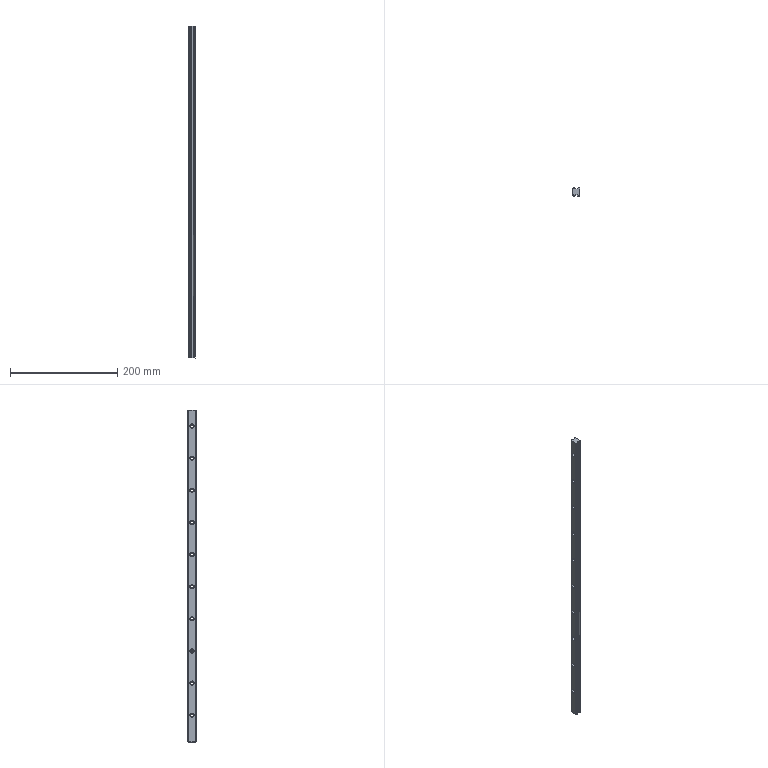Component | SolidWorks | 15x620LinearRail-1 | 1 solid | 83 faces | box 13.17 x 15 x 620.01 mm | volume 96144 mm3 | cylinder 57 | plane 26 | commonest cylinder face diameters 4.8 x20 8 x20 1 x6 0.6 x6 3 x5